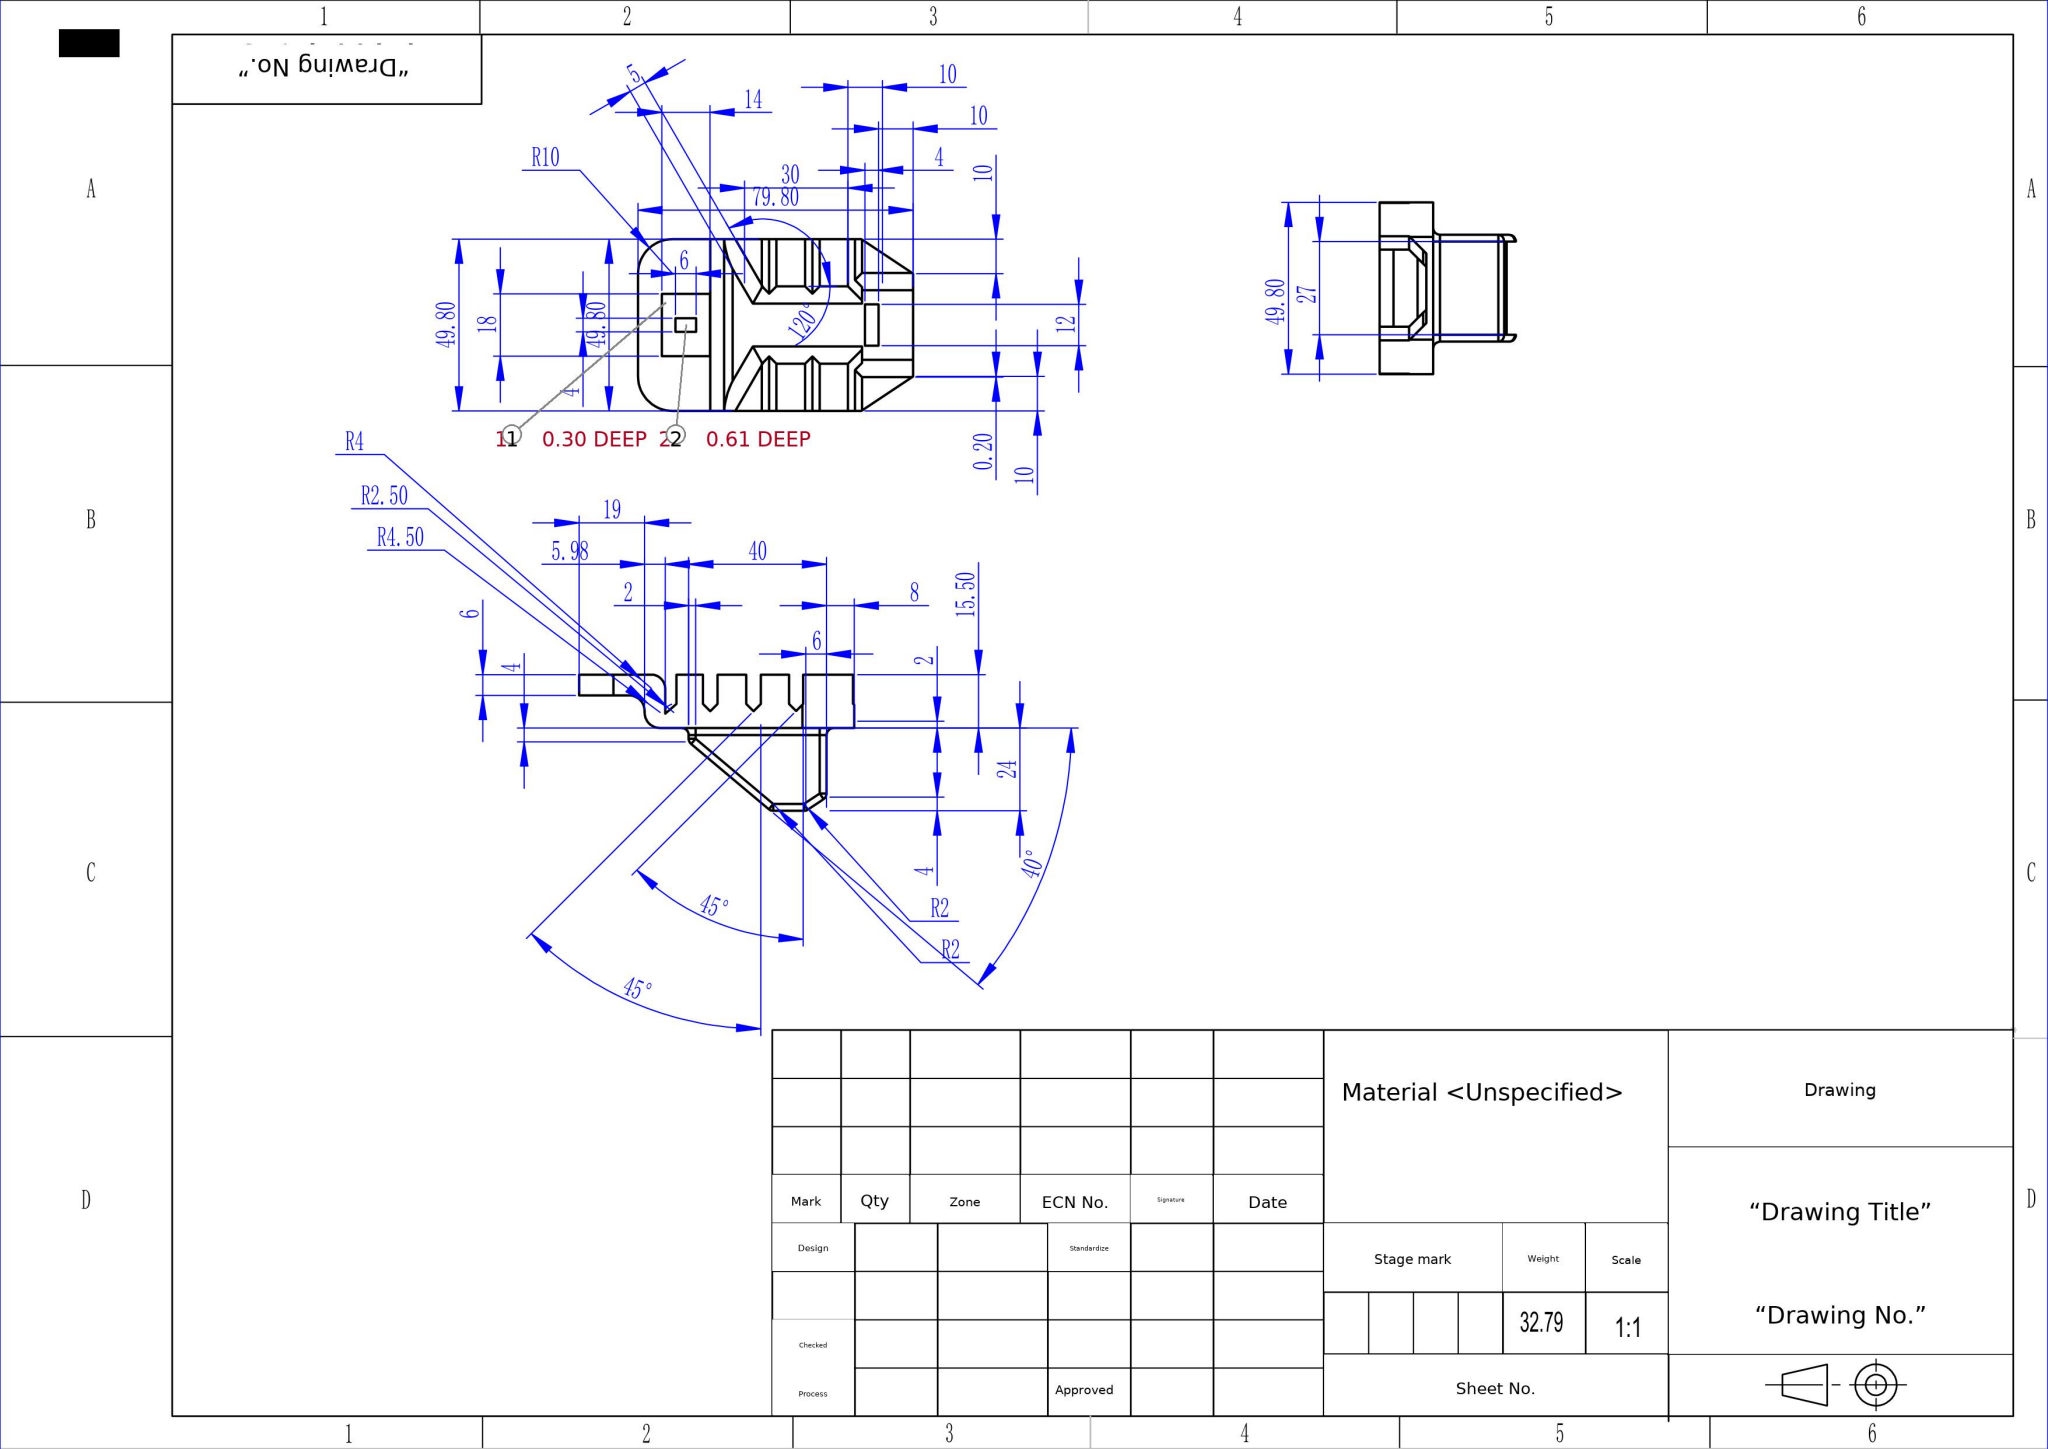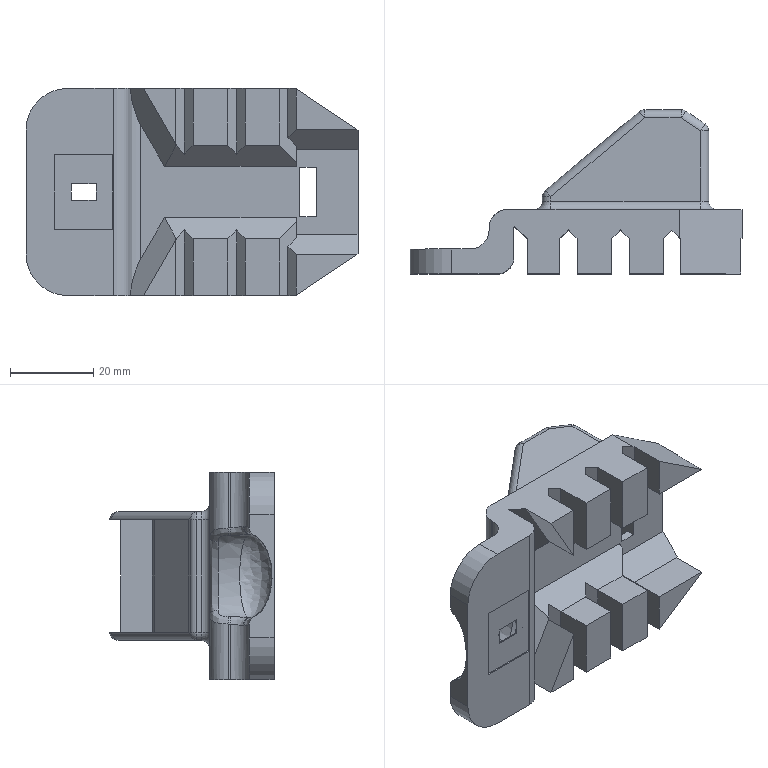Part | SolidWorks | mm | 1 solid | 148 faces | box 79.8 x 39.5 x 49.8 mm | volume 32788 mm3 | plane 95 | cylinder 29 | spline 12 | sphere 8 | torus 4 | commonest cylinder face diameters 4 x21 9 x4 20 x2 5 x1 8 x1